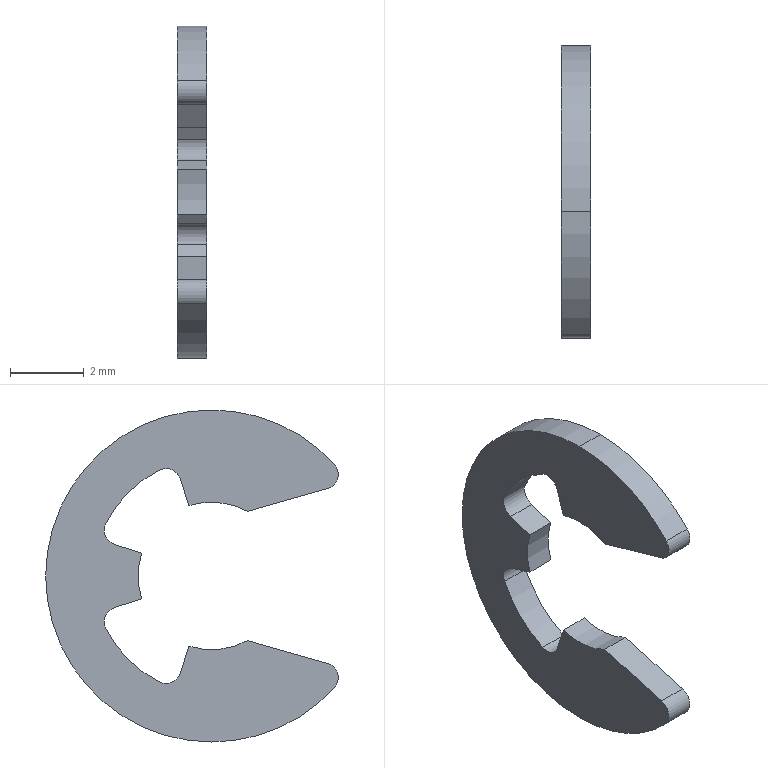Component | SolidWorks | LeverHydraulicRod22-6_e rings gb_GB_CONNECTING_PIECE_RINGS_HR 4-1 | 1 solid | 24 faces | volume 27 mm3 | cylinder 16 | plane 8 | commonest cylinder face diameters 0.8 x7 4 x4 9 x3 6.4 x2